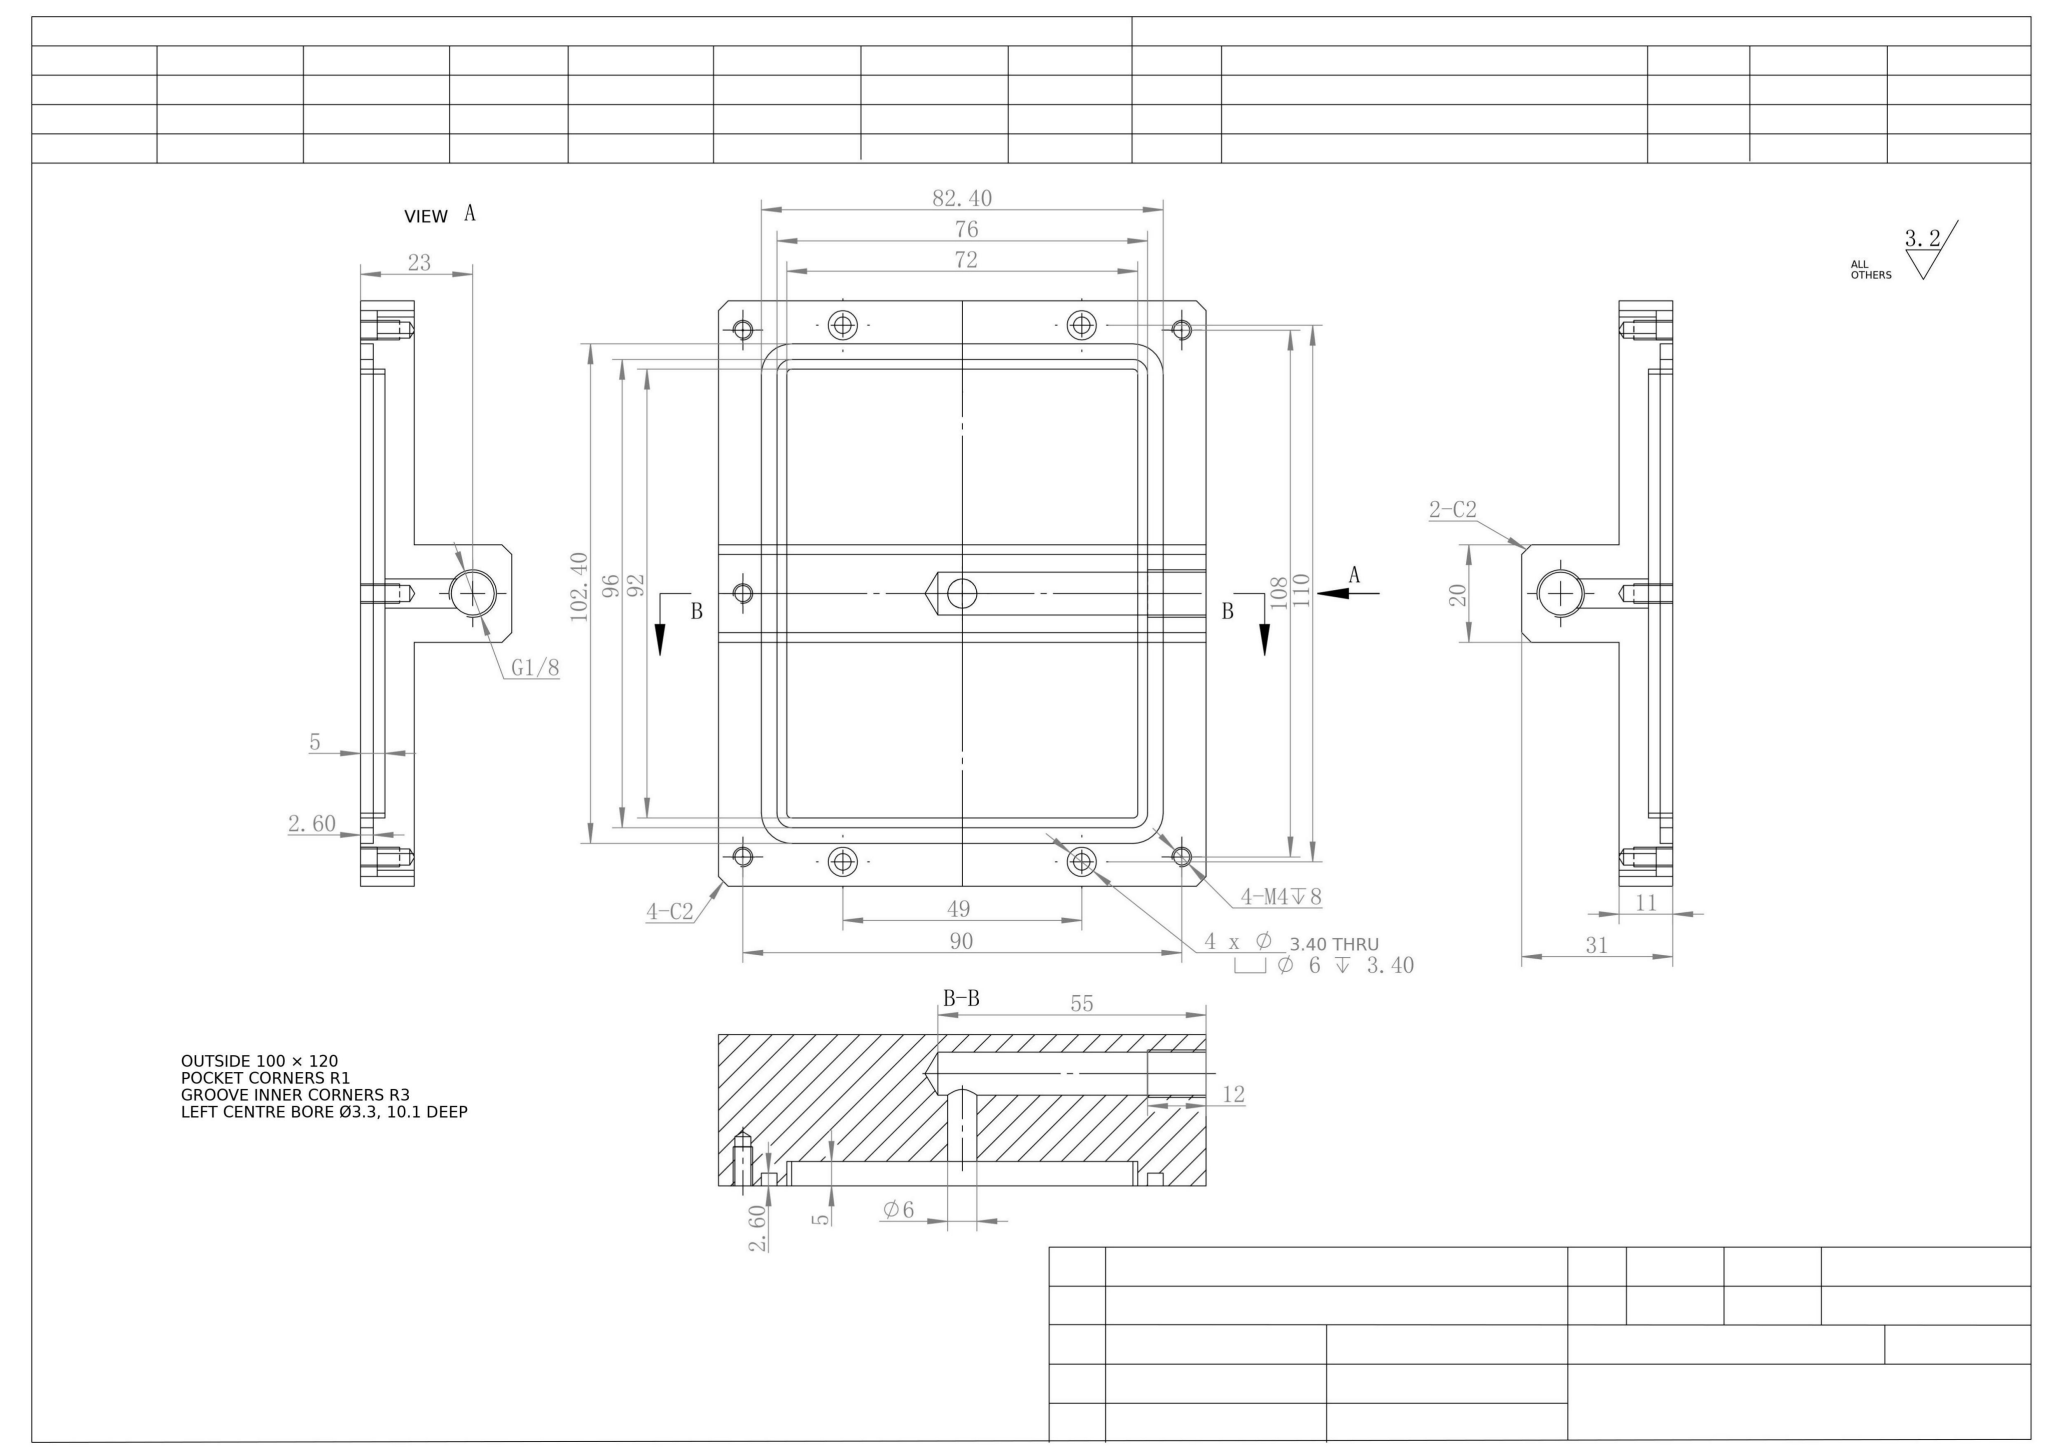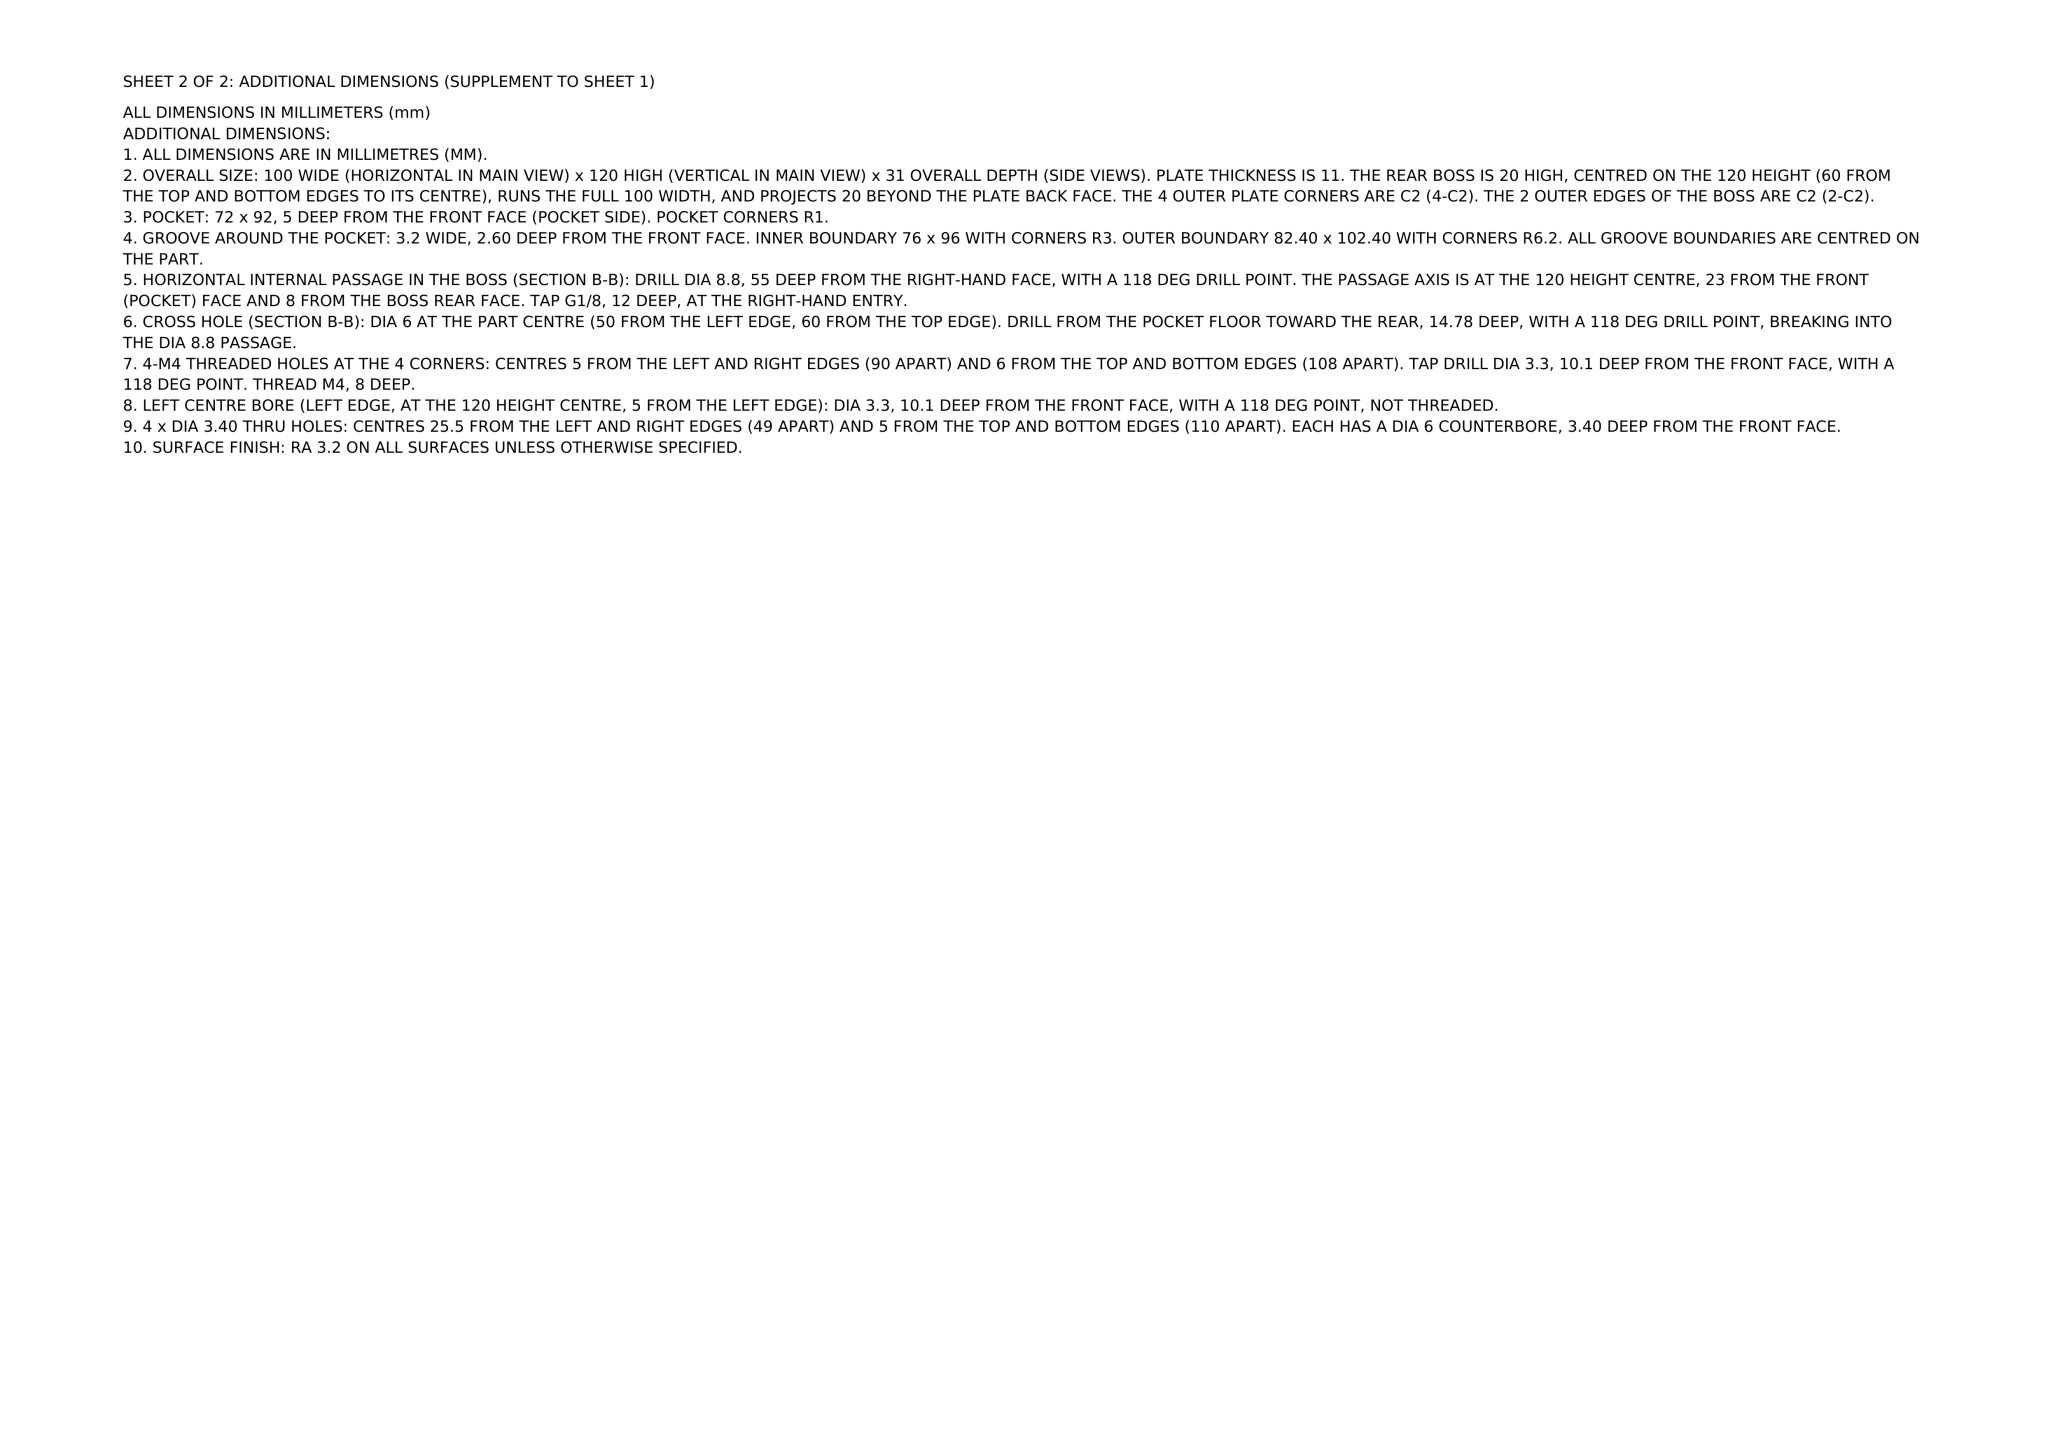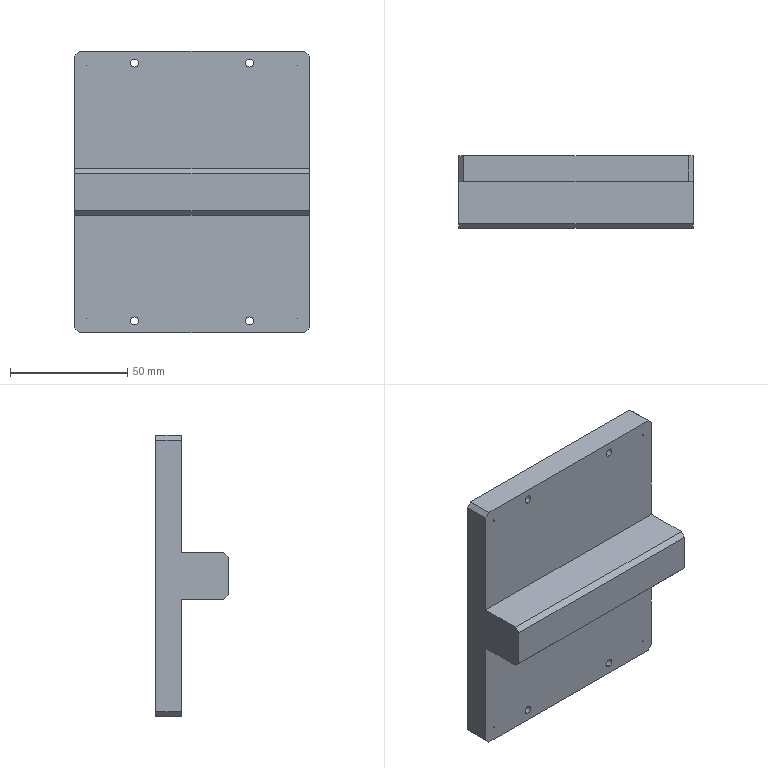Part | NX | mm | Flanged Rectangular Enclosure Housing | 1 solid | 89 faces | box 100 x 31 x 120 mm | volume 130596 mm3 | cylinder 42 | plane 35 | cone 12 | commonest cylinder face diameters 6 x14 3.3 x10 3.4 x8 12.4 x4 2 x4 8.8 x2